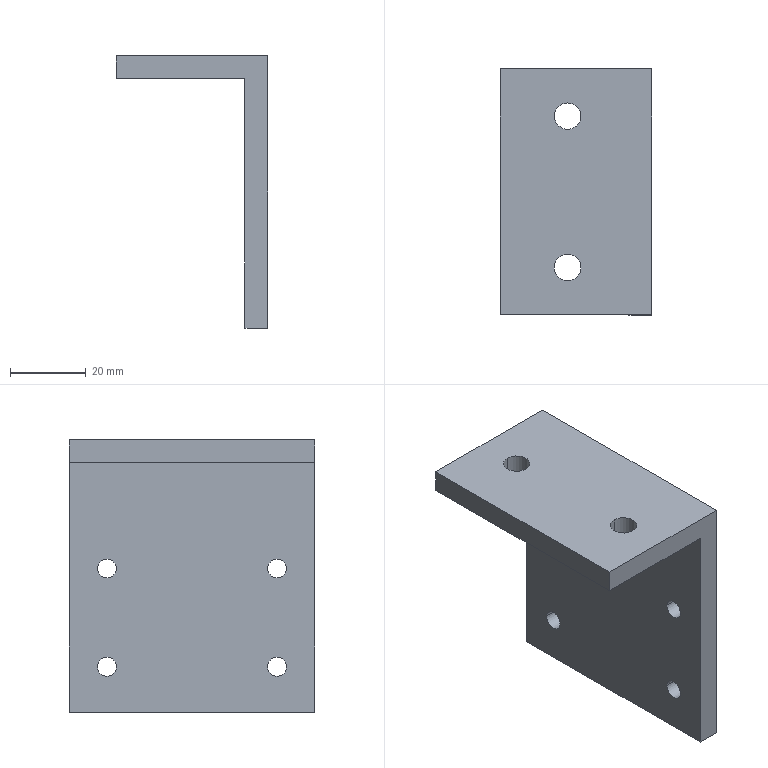Component | SolidWorks | DC-Motor-116-1 | 1 solid | 20 faces | box 40 x 65 x 72 mm | volume 40407 mm3 | cylinder 12 | plane 8 | commonest cylinder face diameters 5 x8 7 x4
build123d program:
from build123d import *

# Parameters (mm, degrees)
BOSS_EXTRUDE1_DEPTH      = 32.5
F_7_0_7_DIAMETER_HOLE1_D = 7
M6_TAPPED_HOLE1_D        = 5


with BuildPart() as part:
    # Sketch1 → Boss-Extrude1 (new, symmetric)
    with BuildSketch(Plane.XY):
        Polygon((-40, 0), (0, 0), (0, 72), (-6, 72), (-6, 6), (-40, 6), align=None)
    extrude(amount=BOSS_EXTRUDE1_DEPTH, both=True)

    # 7.0 _7_ Diameter Hole1 (through all)
    with Locations(Plane(origin=(0, 6, 0), x_dir=(1, 0, 0), z_dir=(0, 1, 0))):
        with Locations((-22.215, 20), (-22.215, -20)):
            Hole(F_7_0_7_DIAMETER_HOLE1_D / 2)

    # M6 Tapped Hole1 (through all)
    with Locations(Plane.ZY.offset(6)):
        with Locations((-22.5, 60), (22.5, 60), (22.5, 34), (-22.5, 34)):
            Hole(M6_TAPPED_HOLE1_D / 2)


solid = part.part

# Placed as in the assembly
solid = solid.moved(Location((-357.792, -173.199, -416), (-90, 0, 0)))
STEP:
#1=COLOUR_RGB('',0.7922,0.8196,0.9333);
#2=FILL_AREA_STYLE_COLOUR('',#1);
#3=FILL_AREA_STYLE('',(#2));
#4=SURFACE_STYLE_FILL_AREA(#3);
#5=SURFACE_SIDE_STYLE('',(#4));
#6=SURFACE_STYLE_USAGE(.BOTH.,#5);
#7=PRESENTATION_STYLE_ASSIGNMENT((#6));
#8=CARTESIAN_POINT('',(-14.086,-7.803,-18.74));
#9=VERTEX_POINT('',#8);
#10=CARTESIAN_POINT('',(-14.086,-7.606,-18.74));
#11=VERTEX_POINT('',#10);
#12=CARTESIAN_POINT('',(-14.086,-7.705,-18.74));
#13=DIRECTION('',(-1.,0.,-0.));
#14=DIRECTION('',(0.,1.,0.));
#15=AXIS2_PLACEMENT_3D('',#12,#13,#14);
#16=CIRCLE('',#15,0.09843);
#17=EDGE_CURVE('',#9,#11,#16,.T.);
#18=ORIENTED_EDGE('',*,*,#17,.F.);
#19=CARTESIAN_POINT('',(-14.323,-7.803,-18.74));
#20=VERTEX_POINT('',#19);
#21=CARTESIAN_POINT('',(-14.323,-7.803,-18.74));
#22=DIRECTION('',(-1.,0.,-0.));
#23=VECTOR('',#22,39.37);
#24=LINE('',#21,#23);
#25=EDGE_CURVE('',#9,#20,#24,.T.);
#26=ORIENTED_EDGE('',*,*,#25,.T.);
#27=CARTESIAN_POINT('',(-14.323,-7.606,-18.74));
#28=VERTEX_POINT('',#27);
#29=CARTESIAN_POINT('',(-14.323,-7.705,-18.74));
#30=DIRECTION('',(-1.,0.,-0.));
#31=DIRECTION('',(0.,1.,0.));
#32=AXIS2_PLACEMENT_3D('',#29,#30,#31);
#33=CIRCLE('',#32,0.09843);
#34=EDGE_CURVE('',#20,#28,#33,.T.);
#35=ORIENTED_EDGE('',*,*,#34,.T.);
#36=CARTESIAN_POINT('',(-14.323,-7.606,-18.74));
#37=DIRECTION('',(-1.,0.,-0.));
#38=VECTOR('',#37,39.37);
#39=LINE('',#36,#38);
#40=EDGE_CURVE('',#11,#28,#39,.T.);
#41=ORIENTED_EDGE('',*,*,#40,.F.);
#42=EDGE_LOOP('',(#18,#26,#35,#41));
#43=FACE_OUTER_BOUND('',#42,.T.);
#44=CARTESIAN_POINT('',(-14.323,-7.705,-18.74));
#45=DIRECTION('',(-1.,0.,-0.));
#46=DIRECTION('',(0.,1.,0.));
#47=AXIS2_PLACEMENT_3D('',#44,#45,#46);
#48=CYLINDRICAL_SURFACE('',#47,0.09843);
#49=ADVANCED_FACE('',(#43),#48,.F.);
#50=CARTESIAN_POINT('',(-14.086,-6.031,-18.74));
#51=VERTEX_POINT('',#50);
#52=CARTESIAN_POINT('',(-14.086,-5.835,-18.74));
#53=VERTEX_POINT('',#52);
#54=CARTESIAN_POINT('',(-14.086,-5.933,-18.74));
#55=DIRECTION('',(-1.,0.,-0.));
#56=DIRECTION('',(0.,1.,0.));
#57=AXIS2_PLACEMENT_3D('',#54,#55,#56);
#58=CIRCLE('',#57,0.09843);
#59=EDGE_CURVE('',#51,#53,#58,.T.);
#60=ORIENTED_EDGE('',*,*,#59,.F.);
#61=CARTESIAN_POINT('',(-14.323,-6.031,-18.74));
#62=VERTEX_POINT('',#61);
#63=CARTESIAN_POINT('',(-14.323,-6.031,-18.74));
#64=DIRECTION('',(-1.,0.,-0.));
#65=VECTOR('',#64,39.37);
#66=LINE('',#63,#65);
#67=EDGE_CURVE('',#51,#62,#66,.T.);
#68=ORIENTED_EDGE('',*,*,#67,.T.);
#69=CARTESIAN_POINT('',(-14.323,-5.835,-18.74));
#70=VERTEX_POINT('',#69);
#71=CARTESIAN_POINT('',(-14.323,-5.933,-18.74));
#72=DIRECTION('',(-1.,0.,-0.));
#73=DIRECTION('',(0.,1.,0.));
#74=AXIS2_PLACEMENT_3D('',#71,#72,#73);
#75=CIRCLE('',#74,0.09843);
#76=EDGE_CURVE('',#62,#70,#75,.T.);
#77=ORIENTED_EDGE('',*,*,#76,.T.);
#78=CARTESIAN_POINT('',(-14.323,-5.835,-18.74));
#79=DIRECTION('',(-1.,0.,-0.));
#80=VECTOR('',#79,39.37);
#81=LINE('',#78,#80);
#82=EDGE_CURVE('',#53,#70,#81,.T.);
#83=ORIENTED_EDGE('',*,*,#82,.F.);
#84=EDGE_LOOP('',(#60,#68,#77,#83));
#85=FACE_OUTER_BOUND('',#84,.T.);
#86=CARTESIAN_POINT('',(-14.323,-5.933,-18.74));
#87=DIRECTION('',(-1.,0.,-0.));
#88=DIRECTION('',(0.,1.,0.));
#89=AXIS2_PLACEMENT_3D('',#86,#87,#88);
#90=CYLINDRICAL_SURFACE('',#89,0.09843);
#91=ADVANCED_FACE('',(#85),#90,.F.);
#92=CARTESIAN_POINT('',(-14.086,-6.031,-17.717));
#93=VERTEX_POINT('',#92);
#94=CARTESIAN_POINT('',(-14.086,-5.835,-17.717));
#95=VERTEX_POINT('',#94);
#96=CARTESIAN_POINT('',(-14.086,-5.933,-17.717));
#97=DIRECTION('',(-1.,0.,-0.));
#98=DIRECTION('',(0.,1.,0.));
#99=AXIS2_PLACEMENT_3D('',#96,#97,#98);
#100=CIRCLE('',#99,0.09843);
#101=EDGE_CURVE('',#93,#95,#100,.T.);
#102=ORIENTED_EDGE('',*,*,#101,.F.);
#103=CARTESIAN_POINT('',(-14.323,-6.031,-17.717));
#104=VERTEX_POINT('',#103);
#105=CARTESIAN_POINT('',(-14.323,-6.031,-17.717));
#106=DIRECTION('',(-1.,0.,-0.));
#107=VECTOR('',#106,39.37);
#108=LINE('',#105,#107);
#109=EDGE_CURVE('',#93,#104,#108,.T.);
#110=ORIENTED_EDGE('',*,*,#109,.T.);
#111=CARTESIAN_POINT('',(-14.323,-5.835,-17.717));
#112=VERTEX_POINT('',#111);
#113=CARTESIAN_POINT('',(-14.323,-5.933,-17.717));
#114=DIRECTION('',(-1.,0.,-0.));
#115=DIRECTION('',(0.,1.,0.));
#116=AXIS2_PLACEMENT_3D('',#113,#114,#115);
#117=CIRCLE('',#116,0.09843);
#118=EDGE_CURVE('',#104,#112,#117,.T.);
#119=ORIENTED_EDGE('',*,*,#118,.T.);
#120=CARTESIAN_POINT('',(-14.323,-5.835,-17.717));
#121=DIRECTION('',(-1.,0.,-0.));
#122=VECTOR('',#121,39.37);
#123=LINE('',#120,#122);
#124=EDGE_CURVE('',#95,#112,#123,.T.);
#125=ORIENTED_EDGE('',*,*,#124,.F.);
#126=EDGE_LOOP('',(#102,#110,#119,#125));
#127=FACE_OUTER_BOUND('',#126,.T.);
#128=CARTESIAN_POINT('',(-14.323,-5.933,-17.717));
#129=DIRECTION('',(-1.,0.,-0.));
#130=DIRECTION('',(0.,1.,0.));
#131=AXIS2_PLACEMENT_3D('',#128,#129,#130);
#132=CYLINDRICAL_SURFACE('',#131,0.09843);
#133=ADVANCED_FACE('',(#127),#132,.F.);
#134=CARTESIAN_POINT('',(-14.086,-7.803,-17.717));
#135=VERTEX_POINT('',#134);
#136=CARTESIAN_POINT('',(-14.086,-7.606,-17.717));
#137=VERTEX_POINT('',#136);
#138=CARTESIAN_POINT('',(-14.086,-7.705,-17.717));
#139=DIRECTION('',(-1.,0.,-0.));
#140=DIRECTION('',(0.,1.,0.));
#141=AXIS2_PLACEMENT_3D('',#138,#139,#140);
#142=CIRCLE('',#141,0.09843);
#143=EDGE_CURVE('',#135,#137,#142,.T.);
#144=ORIENTED_EDGE('',*,*,#143,.F.);
#145=CARTESIAN_POINT('',(-14.323,-7.803,-17.717));
#146=VERTEX_POINT('',#145);
#147=CARTESIAN_POINT('',(-14.323,-7.803,-17.717));
#148=DIRECTION('',(-1.,0.,-0.));
#149=VECTOR('',#148,39.37);
#150=LINE('',#147,#149);
#151=EDGE_CURVE('',#135,#146,#150,.T.);
#152=ORIENTED_EDGE('',*,*,#151,.T.);
#153=CARTESIAN_POINT('',(-14.323,-7.606,-17.717));
#154=VERTEX_POINT('',#153);
#155=CARTESIAN_POINT('',(-14.323,-7.705,-17.717));
#156=DIRECTION('',(-1.,0.,-0.));
#157=DIRECTION('',(0.,1.,0.));
#158=AXIS2_PLACEMENT_3D('',#155,#156,#157);
#159=CIRCLE('',#158,0.09843);
#160=EDGE_CURVE('',#146,#154,#159,.T.);
#161=ORIENTED_EDGE('',*,*,#160,.T.);
#162=CARTESIAN_POINT('',(-14.323,-7.606,-17.717));
#163=DIRECTION('',(-1.,0.,-0.));
#164=VECTOR('',#163,39.37);
#165=LINE('',#162,#164);
#166=EDGE_CURVE('',#137,#154,#165,.T.);
#167=ORIENTED_EDGE('',*,*,#166,.F.);
#168=EDGE_LOOP('',(#144,#152,#161,#167));
#169=FACE_OUTER_BOUND('',#168,.T.);
#170=CARTESIAN_POINT('',(-14.323,-7.705,-17.717));
#171=DIRECTION('',(-1.,0.,-0.));
#172=DIRECTION('',(0.,1.,0.));
#173=AXIS2_PLACEMENT_3D('',#170,#171,#172);
#174=CYLINDRICAL_SURFACE('',#173,0.09843);
#175=ADVANCED_FACE('',(#169),#174,.F.);
#176=CARTESIAN_POINT('',(-14.961,-7.744,-16.378));
#177=VERTEX_POINT('',#176);
#178=CARTESIAN_POINT('',(-14.961,-7.468,-16.378));
#179=VERTEX_POINT('',#178);
#180=CARTESIAN_POINT('',(-14.961,-7.606,-16.378));
#181=DIRECTION('',(0.,0.,-1.));
#182=DIRECTION('',(0.,1.,0.));
#183=AXIS2_PLACEMENT_3D('',#180,#181,#182);
#184=CIRCLE('',#183,0.1378);
#185=EDGE_CURVE('',#177,#179,#184,.T.);
#186=ORIENTED_EDGE('',*,*,#185,.F.);
#187=CARTESIAN_POINT('',(-14.961,-7.744,-16.614));
#188=VERTEX_POINT('',#187);
#189=CARTESIAN_POINT('',(-14.961,-7.744,-16.614));
#190=DIRECTION('',(0.,0.,-1.));
#191=VECTOR('',#190,39.37);
#192=LINE('',#189,#191);
#193=EDGE_CURVE('',#177,#188,#192,.T.);
#194=ORIENTED_EDGE('',*,*,#193,.T.);
#195=CARTESIAN_POINT('',(-14.961,-7.468,-16.614));
#196=VERTEX_POINT('',#195);
#197=CARTESIAN_POINT('',(-14.961,-7.606,-16.614));
#198=DIRECTION('',(0.,0.,-1.));
#199=DIRECTION('',(0.,1.,0.));
#200=AXIS2_PLACEMENT_3D('',#197,#198,#199);
#201=CIRCLE('',#200,0.1378);
#202=EDGE_CURVE('',#188,#196,#201,.T.);
#203=ORIENTED_EDGE('',*,*,#202,.T.);
#204=CARTESIAN_POINT('',(-14.961,-7.468,-16.614));
#205=DIRECTION('',(0.,0.,-1.));
#206=VECTOR('',#205,39.37);
#207=LINE('',#204,#206);
#208=EDGE_CURVE('',#179,#196,#207,.T.);
#209=ORIENTED_EDGE('',*,*,#208,.F.);
#210=EDGE_LOOP('',(#186,#194,#203,#209));
#211=FACE_OUTER_BOUND('',#210,.T.);
#212=CARTESIAN_POINT('',(-14.961,-7.606,-16.614));
#213=DIRECTION('',(0.,0.,-1.));
#214=DIRECTION('',(0.,1.,0.));
#215=AXIS2_PLACEMENT_3D('',#212,#213,#214);
#216=CYLINDRICAL_SURFACE('',#215,0.1378);
#217=ADVANCED_FACE('',(#211),#216,.F.);
#218=CARTESIAN_POINT('',(-14.961,-6.169,-16.378));
#219=VERTEX_POINT('',#218);
#220=CARTESIAN_POINT('',(-14.961,-5.894,-16.378));
#221=VERTEX_POINT('',#220);
#222=CARTESIAN_POINT('',(-14.961,-6.031,-16.378));
#223=DIRECTION('',(0.,0.,-1.));
#224=DIRECTION('',(0.,1.,0.));
#225=AXIS2_PLACEMENT_3D('',#222,#223,#224);
#226=CIRCLE('',#225,0.1378);
#227=EDGE_CURVE('',#219,#221,#226,.T.);
#228=ORIENTED_EDGE('',*,*,#227,.F.);
#229=CARTESIAN_POINT('',(-14.961,-6.169,-16.614));
#230=VERTEX_POINT('',#229);
#231=CARTESIAN_POINT('',(-14.961,-6.169,-16.614));
#232=DIRECTION('',(0.,0.,-1.));
#233=VECTOR('',#232,39.37);
#234=LINE('',#231,#233);
#235=EDGE_CURVE('',#219,#230,#234,.T.);
#236=ORIENTED_EDGE('',*,*,#235,.T.);
#237=CARTESIAN_POINT('',(-14.961,-5.894,-16.614));
#238=VERTEX_POINT('',#237);
#239=CARTESIAN_POINT('',(-14.961,-6.031,-16.614));
#240=DIRECTION('',(0.,0.,-1.));
#241=DIRECTION('',(0.,1.,0.));
#242=AXIS2_PLACEMENT_3D('',#239,#240,#241);
#243=CIRCLE('',#242,0.1378);
#244=EDGE_CURVE('',#230,#238,#243,.T.);
#245=ORIENTED_EDGE('',*,*,#244,.T.);
#246=CARTESIAN_POINT('',(-14.961,-5.894,-16.614));
#247=DIRECTION('',(0.,0.,-1.));
#248=VECTOR('',#247,39.37);
#249=LINE('',#246,#248);
#250=EDGE_CURVE('',#221,#238,#249,.T.);
#251=ORIENTED_EDGE('',*,*,#250,.F.);
#252=EDGE_LOOP('',(#228,#236,#245,#251));
#253=FACE_OUTER_BOUND('',#252,.T.);
#254=CARTESIAN_POINT('',(-14.961,-6.031,-16.614));
#255=DIRECTION('',(0.,0.,-1.));
#256=DIRECTION('',(0.,1.,0.));
#257=AXIS2_PLACEMENT_3D('',#254,#255,#256);
#258=CYLINDRICAL_SURFACE('',#257,0.1378);
#259=ADVANCED_FACE('',(#253),#258,.F.);
#260=CARTESIAN_POINT('',(-15.661,-8.098,-16.614));
#261=VERTEX_POINT('',#260);
#262=CARTESIAN_POINT('',(-15.661,-8.098,-16.378));
#263=VERTEX_POINT('',#262);
#264=CARTESIAN_POINT('',(-15.661,-8.098,-16.614));
#265=DIRECTION('',(-0.,-0.,1.));
#266=VECTOR('',#265,39.37);
#267=LINE('',#264,#266);
#268=EDGE_CURVE('',#261,#263,#267,.T.);
#269=ORIENTED_EDGE('',*,*,#268,.T.);
#270=CARTESIAN_POINT('',(-15.661,-5.539,-16.378));
#271=VERTEX_POINT('',#270);
#272=CARTESIAN_POINT('',(-15.661,-5.539,-16.378));
#273=DIRECTION('',(-0.,-1.,-0.));
#274=VECTOR('',#273,39.37);
#275=LINE('',#272,#274);
#276=EDGE_CURVE('',#271,#263,#275,.T.);
#277=ORIENTED_EDGE('',*,*,#276,.F.);
#278=CARTESIAN_POINT('',(-15.661,-5.539,-16.614));
#279=VERTEX_POINT('',#278);
#280=CARTESIAN_POINT('',(-15.661,-5.539,-16.614));
#281=DIRECTION('',(-0.,-0.,1.));
#282=VECTOR('',#281,39.37);
#283=LINE('',#280,#282);
#284=EDGE_CURVE('',#279,#271,#283,.T.);
#285=ORIENTED_EDGE('',*,*,#284,.F.);
#286=CARTESIAN_POINT('',(-15.661,-5.539,-16.614));
#287=DIRECTION('',(-0.,-1.,-0.));
#288=VECTOR('',#287,39.37);
#289=LINE('',#286,#288);
#290=EDGE_CURVE('',#279,#261,#289,.T.);
#291=ORIENTED_EDGE('',*,*,#290,.T.);
#292=EDGE_LOOP('',(#269,#277,#285,#291));
#293=FACE_OUTER_BOUND('',#292,.T.);
#294=CARTESIAN_POINT('',(-15.661,-5.539,-16.614));
#295=DIRECTION('',(1.,-0.,0.));
#296=DIRECTION('',(-0.,-1.,-0.));
#297=AXIS2_PLACEMENT_3D('',#294,#295,#296);
#298=PLANE('',#297);
#299=ADVANCED_FACE('',(#293),#298,.F.);
#300=CARTESIAN_POINT('',(-14.961,-7.606,-16.378));
#301=DIRECTION('',(0.,0.,-1.));
#302=DIRECTION('',(0.,1.,0.));
#303=AXIS2_PLACEMENT_3D('',#300,#301,#302);
#304=CIRCLE('',#303,0.1378);
#305=EDGE_CURVE('',#179,#177,#304,.T.);
#306=ORIENTED_EDGE('',*,*,#305,.T.);
#307=ORIENTED_EDGE('',*,*,#185,.T.);
#308=EDGE_LOOP('',(#306,#307));
#309=FACE_BOUND('',#308,.T.);
#310=CARTESIAN_POINT('',(-14.961,-6.031,-16.378));
#311=DIRECTION('',(0.,0.,-1.));
#312=DIRECTION('',(0.,1.,0.));
#313=AXIS2_PLACEMENT_3D('',#310,#311,#312);
#314=CIRCLE('',#313,0.1378);
#315=EDGE_CURVE('',#221,#219,#314,.T.);
#316=ORIENTED_EDGE('',*,*,#315,.T.);
#317=ORIENTED_EDGE('',*,*,#227,.T.);
#318=EDGE_LOOP('',(#316,#317));
#319=FACE_BOUND('',#318,.T.);
#320=CARTESIAN_POINT('',(-14.086,-8.098,-16.378));
#321=VERTEX_POINT('',#320);
#322=CARTESIAN_POINT('',(-15.661,-8.098,-16.378));
#323=DIRECTION('',(1.,-0.,0.));
#324=VECTOR('',#323,39.37);
#325=LINE('',#322,#324);
#326=EDGE_CURVE('',#263,#321,#325,.T.);
#327=ORIENTED_EDGE('',*,*,#326,.T.);
#328=CARTESIAN_POINT('',(-14.086,-5.539,-16.378));
#329=VERTEX_POINT('',#328);
#330=CARTESIAN_POINT('',(-14.086,-5.539,-16.378));
#331=DIRECTION('',(-0.,-1.,-0.));
#332=VECTOR('',#331,39.37);
#333=LINE('',#330,#332);
#334=EDGE_CURVE('',#329,#321,#333,.T.);
#335=ORIENTED_EDGE('',*,*,#334,.F.);
#336=CARTESIAN_POINT('',(-15.661,-5.539,-16.378));
#337=DIRECTION('',(1.,-0.,0.));
#338=VECTOR('',#337,39.37);
#339=LINE('',#336,#338);
#340=EDGE_CURVE('',#271,#329,#339,.T.);
#341=ORIENTED_EDGE('',*,*,#340,.F.);
#342=ORIENTED_EDGE('',*,*,#276,.T.);
#343=EDGE_LOOP('',(#327,#335,#341,#342));
#344=FACE_OUTER_BOUND('',#343,.T.);
#345=CARTESIAN_POINT('',(-15.661,-5.539,-16.378));
#346=DIRECTION('',(0.,0.,-1.));
#347=DIRECTION('',(0.,1.,0.));
#348=AXIS2_PLACEMENT_3D('',#345,#346,#347);
#349=PLANE('',#348);
#350=ADVANCED_FACE('',(#309,#319,#344),#349,.F.);
#351=CARTESIAN_POINT('',(-14.086,-7.705,-18.74));
#352=DIRECTION('',(-1.,0.,-0.));
#353=DIRECTION('',(0.,1.,0.));
#354=AXIS2_PLACEMENT_3D('',#351,#352,#353);
#355=CIRCLE('',#354,0.09843);
#356=EDGE_CURVE('',#11,#9,#355,.T.);
#357=ORIENTED_EDGE('',*,*,#356,.T.);
#358=ORIENTED_EDGE('',*,*,#17,.T.);
#359=EDGE_LOOP('',(#357,#358));
#360=FACE_BOUND('',#359,.T.);
#361=CARTESIAN_POINT('',(-14.086,-5.933,-18.74));
#362=DIRECTION('',(-1.,0.,-0.));
#363=DIRECTION('',(0.,1.,0.));
#364=AXIS2_PLACEMENT_3D('',#361,#362,#363);
#365=CIRCLE('',#364,0.09843);
#366=EDGE_CURVE('',#53,#51,#365,.T.);
#367=ORIENTED_EDGE('',*,*,#366,.T.);
#368=ORIENTED_EDGE('',*,*,#59,.T.);
#369=EDGE_LOOP('',(#367,#368));
#370=FACE_BOUND('',#369,.T.);
#371=CARTESIAN_POINT('',(-14.086,-5.933,-17.717));
#372=DIRECTION('',(-1.,0.,-0.));
#373=DIRECTION('',(0.,1.,0.));
#374=AXIS2_PLACEMENT_3D('',#371,#372,#373);
#375=CIRCLE('',#374,0.09843);
#376=EDGE_CURVE('',#95,#93,#375,.T.);
#377=ORIENTED_EDGE('',*,*,#376,.T.);
#378=ORIENTED_EDGE('',*,*,#101,.T.);
#379=EDGE_LOOP('',(#377,#378));
#380=FACE_BOUND('',#379,.T.);
#381=CARTESIAN_POINT('',(-14.086,-7.705,-17.717));
#382=DIRECTION('',(-1.,0.,-0.));
#383=DIRECTION('',(0.,1.,0.));
#384=AXIS2_PLACEMENT_3D('',#381,#382,#383);
#385=CIRCLE('',#384,0.09843);
#386=EDGE_CURVE('',#137,#135,#385,.T.);
#387=ORIENTED_EDGE('',*,*,#386,.T.);
#388=ORIENTED_EDGE('',*,*,#143,.T.);
#389=EDGE_LOOP('',(#387,#388));
#390=FACE_BOUND('',#389,.T.);
#391=CARTESIAN_POINT('',(-14.086,-8.098,-19.213));
#392=VERTEX_POINT('',#391);
#393=CARTESIAN_POINT('',(-14.086,-8.098,-16.378));
#394=DIRECTION('',(0.,0.,-1.));
#395=VECTOR('',#394,39.37);
#396=LINE('',#393,#395);
#397=EDGE_CURVE('',#321,#392,#396,.T.);
#398=ORIENTED_EDGE('',*,*,#397,.T.);
#399=CARTESIAN_POINT('',(-14.086,-5.539,-19.213));
#400=VERTEX_POINT('',#399);
#401=CARTESIAN_POINT('',(-14.086,-5.539,-19.213));
#402=DIRECTION('',(-0.,-1.,-0.));
#403=VECTOR('',#402,39.37);
#404=LINE('',#401,#403);
#405=EDGE_CURVE('',#400,#392,#404,.T.);
#406=ORIENTED_EDGE('',*,*,#405,.F.);
#407=CARTESIAN_POINT('',(-14.086,-5.539,-16.378));
#408=DIRECTION('',(0.,0.,-1.));
#409=VECTOR('',#408,39.37);
#410=LINE('',#407,#409);
#411=EDGE_CURVE('',#329,#400,#410,.T.);
#412=ORIENTED_EDGE('',*,*,#411,.F.);
#413=ORIENTED_EDGE('',*,*,#334,.T.);
#414=EDGE_LOOP('',(#398,#406,#412,#413));
#415=FACE_OUTER_BOUND('',#414,.T.);
#416=CARTESIAN_POINT('',(-14.086,-5.539,-16.378));
#417=DIRECTION('',(-1.,0.,-0.));
#418=DIRECTION('',(0.,1.,0.));
#419=AXIS2_PLACEMENT_3D('',#416,#417,#418);
#420=PLANE('',#419);
#421=ADVANCED_FACE('',(#360,#370,#380,#390,#415),#420,.F.);
#422=CARTESIAN_POINT('',(-14.323,-8.098,-19.213));
#423=VERTEX_POINT('',#422);
#424=CARTESIAN_POINT('',(-14.323,-8.098,-19.213));
#425=DIRECTION('',(-1.,0.,-0.));
#426=VECTOR('',#425,39.37);
#427=LINE('',#424,#426);
#428=EDGE_CURVE('',#392,#423,#427,.T.);
#429=ORIENTED_EDGE('',*,*,#428,.T.);
#430=CARTESIAN_POINT('',(-14.323,-5.539,-19.213));
#431=VERTEX_POINT('',#430);
#432=CARTESIAN_POINT('',(-14.323,-5.539,-19.213));
#433=DIRECTION('',(-0.,-1.,-0.));
#434=VECTOR('',#433,39.37);
#435=LINE('',#432,#434);
#436=EDGE_CURVE('',#431,#423,#435,.T.);
#437=ORIENTED_EDGE('',*,*,#436,.F.);
#438=CARTESIAN_POINT('',(-14.323,-5.539,-19.213));
#439=DIRECTION('',(-1.,0.,-0.));
#440=VECTOR('',#439,39.37);
#441=LINE('',#438,#440);
#442=EDGE_CURVE('',#400,#431,#441,.T.);
#443=ORIENTED_EDGE('',*,*,#442,.F.);
#444=ORIENTED_EDGE('',*,*,#405,.T.);
#445=EDGE_LOOP('',(#429,#437,#443,#444));
#446=FACE_OUTER_BOUND('',#445,.T.);
#447=CARTESIAN_POINT('',(-14.323,-5.539,-19.213));
#448=DIRECTION('',(-0.,-0.,1.));
#449=DIRECTION('',(-0.,-1.,-0.));
#450=AXIS2_PLACEMENT_3D('',#447,#448,#449);
#451=PLANE('',#450);
#452=ADVANCED_FACE('',(#446),#451,.F.);
#453=CARTESIAN_POINT('',(-14.323,-7.705,-18.74));
#454=DIRECTION('',(-1.,0.,-0.));
#455=DIRECTION('',(0.,1.,0.));
#456=AXIS2_PLACEMENT_3D('',#453,#454,#455);
#457=CIRCLE('',#456,0.09843);
#458=EDGE_CURVE('',#28,#20,#457,.T.);
#459=ORIENTED_EDGE('',*,*,#458,.F.);
#460=ORIENTED_EDGE('',*,*,#34,.F.);
#461=EDGE_LOOP('',(#459,#460));
#462=FACE_BOUND('',#461,.T.);
#463=CARTESIAN_POINT('',(-14.323,-5.933,-18.74));
#464=DIRECTION('',(-1.,0.,-0.));
#465=DIRECTION('',(0.,1.,0.));
#466=AXIS2_PLACEMENT_3D('',#463,#464,#465);
#467=CIRCLE('',#466,0.09843);
#468=EDGE_CURVE('',#70,#62,#467,.T.);
#469=ORIENTED_EDGE('',*,*,#468,.F.);
#470=ORIENTED_EDGE('',*,*,#76,.F.);
#471=EDGE_LOOP('',(#469,#470));
#472=FACE_BOUND('',#471,.T.);
#473=CARTESIAN_POINT('',(-14.323,-5.933,-17.717));
#474=DIRECTION('',(-1.,0.,-0.));
#475=DIRECTION('',(0.,1.,0.));
#476=AXIS2_PLACEMENT_3D('',#473,#474,#475);
#477=CIRCLE('',#476,0.09843);
#478=EDGE_CURVE('',#112,#104,#477,.T.);
#479=ORIENTED_EDGE('',*,*,#478,.F.);
#480=ORIENTED_EDGE('',*,*,#118,.F.);
#481=EDGE_LOOP('',(#479,#480));
#482=FACE_BOUND('',#481,.T.);
#483=CARTESIAN_POINT('',(-14.323,-7.705,-17.717));
#484=DIRECTION('',(-1.,0.,-0.));
#485=DIRECTION('',(0.,1.,0.));
#486=AXIS2_PLACEMENT_3D('',#483,#484,#485);
#487=CIRCLE('',#486,0.09843);
#488=EDGE_CURVE('',#154,#146,#487,.T.);
#489=ORIENTED_EDGE('',*,*,#488,.F.);
#490=ORIENTED_EDGE('',*,*,#160,.F.);
#491=EDGE_LOOP('',(#489,#490));
#492=FACE_BOUND('',#491,.T.);
#493=CARTESIAN_POINT('',(-14.323,-8.098,-16.614));
#494=VERTEX_POINT('',#493);
#495=CARTESIAN_POINT('',(-14.323,-8.098,-16.614));
#496=DIRECTION('',(-0.,-0.,1.));
#497=VECTOR('',#496,39.37);
#498=LINE('',#495,#497);
#499=EDGE_CURVE('',#423,#494,#498,.T.);
#500=ORIENTED_EDGE('',*,*,#499,.T.);
#501=CARTESIAN_POINT('',(-14.323,-5.539,-16.614));
#502=VERTEX_POINT('',#501);
#503=CARTESIAN_POINT('',(-14.323,-5.539,-16.614));
#504=DIRECTION('',(-0.,-1.,-0.));
#505=VECTOR('',#504,39.37);
#506=LINE('',#503,#505);
#507=EDGE_CURVE('',#502,#494,#506,.T.);
#508=ORIENTED_EDGE('',*,*,#507,.F.);
#509=CARTESIAN_POINT('',(-14.323,-5.539,-16.614));
#510=DIRECTION('',(-0.,-0.,1.));
#511=VECTOR('',#510,39.37);
#512=LINE('',#509,#511);
#513=EDGE_CURVE('',#431,#502,#512,.T.);
#514=ORIENTED_EDGE('',*,*,#513,.F.);
#515=ORIENTED_EDGE('',*,*,#436,.T.);
#516=EDGE_LOOP('',(#500,#508,#514,#515));
#517=FACE_OUTER_BOUND('',#516,.T.);
#518=CARTESIAN_POINT('',(-14.323,-5.539,-16.614));
#519=DIRECTION('',(1.,-0.,0.));
#520=DIRECTION('',(-0.,-1.,-0.));
#521=AXIS2_PLACEMENT_3D('',#518,#519,#520);
#522=PLANE('',#521);
#523=ADVANCED_FACE('',(#462,#472,#482,#492,#517),#522,.F.);
#524=CARTESIAN_POINT('',(-14.961,-7.606,-16.614));
#525=DIRECTION('',(0.,0.,-1.));
#526=DIRECTION('',(0.,1.,0.));
#527=AXIS2_PLACEMENT_3D('',#524,#525,#526);
#528=CIRCLE('',#527,0.1378);
#529=EDGE_CURVE('',#196,#188,#528,.T.);
#530=ORIENTED_EDGE('',*,*,#529,.F.);
#531=ORIENTED_EDGE('',*,*,#202,.F.);
#532=EDGE_LOOP('',(#530,#531));
#533=FACE_BOUND('',#532,.T.);
#534=CARTESIAN_POINT('',(-14.961,-6.031,-16.614));
#535=DIRECTION('',(0.,0.,-1.));
#536=DIRECTION('',(0.,1.,0.));
#537=AXIS2_PLACEMENT_3D('',#534,#535,#536);
#538=CIRCLE('',#537,0.1378);
#539=EDGE_CURVE('',#238,#230,#538,.T.);
#540=ORIENTED_EDGE('',*,*,#539,.F.);
#541=ORIENTED_EDGE('',*,*,#244,.F.);
#542=EDGE_LOOP('',(#540,#541));
#543=FACE_BOUND('',#542,.T.);
#544=CARTESIAN_POINT('',(-15.661,-8.098,-16.614));
#545=DIRECTION('',(-1.,0.,-0.));
#546=VECTOR('',#545,39.37);
#547=LINE('',#544,#546);
#548=EDGE_CURVE('',#494,#261,#547,.T.);
#549=ORIENTED_EDGE('',*,*,#548,.T.);
#550=ORIENTED_EDGE('',*,*,#290,.F.);
#551=CARTESIAN_POINT('',(-15.661,-5.539,-16.614));
#552=DIRECTION('',(-1.,0.,-0.));
#553=VECTOR('',#552,39.37);
#554=LINE('',#551,#553);
#555=EDGE_CURVE('',#502,#279,#554,.T.);
#556=ORIENTED_EDGE('',*,*,#555,.F.);
#557=ORIENTED_EDGE('',*,*,#507,.T.);
#558=EDGE_LOOP('',(#549,#550,#556,#557));
#559=FACE_OUTER_BOUND('',#558,.T.);
#560=CARTESIAN_POINT('',(-15.661,-5.539,-16.614));
#561=DIRECTION('',(-0.,-0.,1.));
#562=DIRECTION('',(-0.,-1.,-0.));
#563=AXIS2_PLACEMENT_3D('',#560,#561,#562);
#564=PLANE('',#563);
#565=ADVANCED_FACE('',(#533,#543,#559),#564,.F.);
#566=ORIENTED_EDGE('',*,*,#284,.T.);
#567=ORIENTED_EDGE('',*,*,#340,.T.);
#568=ORIENTED_EDGE('',*,*,#411,.T.);
#569=ORIENTED_EDGE('',*,*,#442,.T.);
#570=ORIENTED_EDGE('',*,*,#513,.T.);
#571=ORIENTED_EDGE('',*,*,#555,.T.);
#572=EDGE_LOOP('',(#566,#567,#568,#569,#570,#571));
#573=FACE_OUTER_BOUND('',#572,.T.);
#574=CARTESIAN_POINT('',(-14.086,-5.539,-16.378));
#575=DIRECTION('',(0.,1.,0.));
#576=DIRECTION('',(1.,-0.,0.));
#577=AXIS2_PLACEMENT_3D('',#574,#575,#576);
#578=PLANE('',#577);
#579=ADVANCED_FACE('',(#573),#578,.T.);
#580=ORIENTED_EDGE('',*,*,#268,.F.);
#581=ORIENTED_EDGE('',*,*,#548,.F.);
#582=ORIENTED_EDGE('',*,*,#499,.F.);
#583=ORIENTED_EDGE('',*,*,#428,.F.);
#584=ORIENTED_EDGE('',*,*,#397,.F.);
#585=ORIENTED_EDGE('',*,*,#326,.F.);
#586=EDGE_LOOP('',(#580,#581,#582,#583,#584,#585));
#587=FACE_OUTER_BOUND('',#586,.T.);
#588=CARTESIAN_POINT('',(-14.086,-8.098,-16.378));
#589=DIRECTION('',(0.,1.,0.));
#590=DIRECTION('',(1.,-0.,0.));
#591=AXIS2_PLACEMENT_3D('',#588,#589,#590);
#592=PLANE('',#591);
#593=ADVANCED_FACE('',(#587),#592,.F.);
#594=ORIENTED_EDGE('',*,*,#235,.F.);
#595=ORIENTED_EDGE('',*,*,#315,.F.);
#596=ORIENTED_EDGE('',*,*,#250,.T.);
#597=ORIENTED_EDGE('',*,*,#539,.T.);
#598=EDGE_LOOP('',(#594,#595,#596,#597));
#599=FACE_OUTER_BOUND('',#598,.T.);
#600=CARTESIAN_POINT('',(-14.961,-6.031,-16.614));
#601=DIRECTION('',(0.,0.,-1.));
#602=DIRECTION('',(0.,1.,0.));
#603=AXIS2_PLACEMENT_3D('',#600,#601,#602);
#604=CYLINDRICAL_SURFACE('',#603,0.1378);
#605=ADVANCED_FACE('',(#599),#604,.F.);
#606=ORIENTED_EDGE('',*,*,#193,.F.);
#607=ORIENTED_EDGE('',*,*,#305,.F.);
#608=ORIENTED_EDGE('',*,*,#208,.T.);
#609=ORIENTED_EDGE('',*,*,#529,.T.);
#610=EDGE_LOOP('',(#606,#607,#608,#609));
#611=FACE_OUTER_BOUND('',#610,.T.);
#612=CARTESIAN_POINT('',(-14.961,-7.606,-16.614));
#613=DIRECTION('',(0.,0.,-1.));
#614=DIRECTION('',(0.,1.,0.));
#615=AXIS2_PLACEMENT_3D('',#612,#613,#614);
#616=CYLINDRICAL_SURFACE('',#615,0.1378);
#617=ADVANCED_FACE('',(#611),#616,.F.);
#618=ORIENTED_EDGE('',*,*,#151,.F.);
#619=ORIENTED_EDGE('',*,*,#386,.F.);
#620=ORIENTED_EDGE('',*,*,#166,.T.);
#621=ORIENTED_EDGE('',*,*,#488,.T.);
#622=EDGE_LOOP('',(#618,#619,#620,#621));
#623=FACE_OUTER_BOUND('',#622,.T.);
#624=CARTESIAN_POINT('',(-14.323,-7.705,-17.717));
#625=DIRECTION('',(-1.,0.,-0.));
#626=DIRECTION('',(0.,1.,0.));
#627=AXIS2_PLACEMENT_3D('',#624,#625,#626);
#628=CYLINDRICAL_SURFACE('',#627,0.09843);
#629=ADVANCED_FACE('',(#623),#628,.F.);
#630=ORIENTED_EDGE('',*,*,#109,.F.);
#631=ORIENTED_EDGE('',*,*,#376,.F.);
#632=ORIENTED_EDGE('',*,*,#124,.T.);
#633=ORIENTED_EDGE('',*,*,#478,.T.);
#634=EDGE_LOOP('',(#630,#631,#632,#633));
#635=FACE_OUTER_BOUND('',#634,.T.);
#636=CARTESIAN_POINT('',(-14.323,-5.933,-17.717));
#637=DIRECTION('',(-1.,0.,-0.));
#638=DIRECTION('',(0.,1.,0.));
#639=AXIS2_PLACEMENT_3D('',#636,#637,#638);
#640=CYLINDRICAL_SURFACE('',#639,0.09843);
#641=ADVANCED_FACE('',(#635),#640,.F.);
#642=ORIENTED_EDGE('',*,*,#67,.F.);
#643=ORIENTED_EDGE('',*,*,#366,.F.);
#644=ORIENTED_EDGE('',*,*,#82,.T.);
#645=ORIENTED_EDGE('',*,*,#468,.T.);
#646=EDGE_LOOP('',(#642,#643,#644,#645));
#647=FACE_OUTER_BOUND('',#646,.T.);
#648=CARTESIAN_POINT('',(-14.323,-5.933,-18.74));
#649=DIRECTION('',(-1.,0.,-0.));
#650=DIRECTION('',(0.,1.,0.));
#651=AXIS2_PLACEMENT_3D('',#648,#649,#650);
#652=CYLINDRICAL_SURFACE('',#651,0.09843);
#653=ADVANCED_FACE('',(#647),#652,.F.);
#654=ORIENTED_EDGE('',*,*,#25,.F.);
#655=ORIENTED_EDGE('',*,*,#356,.F.);
#656=ORIENTED_EDGE('',*,*,#40,.T.);
#657=ORIENTED_EDGE('',*,*,#458,.T.);
#658=EDGE_LOOP('',(#654,#655,#656,#657));
#659=FACE_OUTER_BOUND('',#658,.T.);
#660=CARTESIAN_POINT('',(-14.323,-7.705,-18.74));
#661=DIRECTION('',(-1.,0.,-0.));
#662=DIRECTION('',(0.,1.,0.));
#663=AXIS2_PLACEMENT_3D('',#660,#661,#662);
#664=CYLINDRICAL_SURFACE('',#663,0.09843);
#665=ADVANCED_FACE('',(#659),#664,.F.);
#666=CLOSED_SHELL('',(#49,#91,#133,#175,#217,#259,#299,#350,#421,#452,#523,#565,#579,#593,#605,#617,#629,#641,#653,#665));
#667=MANIFOLD_SOLID_BREP('',#666);
#668=STYLED_ITEM('',(#7),#667);
#669=(LENGTH_UNIT()NAMED_UNIT(*)SI_UNIT($,.METRE.));
#670=LENGTH_MEASURE_WITH_UNIT(LENGTH_MEASURE(0.0254),#669);
#671=DIMENSIONAL_EXPONENTS(1.,0.,0.,0.,0.,0.,0.);
#672=(CONVERSION_BASED_UNIT('',#670)LENGTH_UNIT()NAMED_UNIT(#671));
#673=UNCERTAINTY_MEASURE_WITH_UNIT(LENGTH_MEASURE(0.00001),#672,'','');
#674=(NAMED_UNIT(*)PLANE_ANGLE_UNIT()SI_UNIT($,.RADIAN.));
#675=(NAMED_UNIT(*)SI_UNIT($,.STERADIAN.)SOLID_ANGLE_UNIT());
#676=(GEOMETRIC_REPRESENTATION_CONTEXT(3)GLOBAL_UNCERTAINTY_ASSIGNED_CONTEXT((#673))GLOBAL_UNIT_ASSIGNED_CONTEXT((#672,#674,#675))REPRESENTATION_CONTEXT('',''));
#677=MECHANICAL_DESIGN_GEOMETRIC_PRESENTATION_REPRESENTATION('',(#668),#676);
#678=PRESENTATION_LAYER_ASSIGNMENT('','',(#668));
#679=CARTESIAN_POINT('',(0.,0.,0.));
#680=DIRECTION('',(0.,0.,1.));
#681=DIRECTION('',(1.,0.,0.));
#682=AXIS2_PLACEMENT_3D('',#679,#680,#681);
#683=(LENGTH_UNIT()NAMED_UNIT(*)SI_UNIT($,.METRE.));
#684=LENGTH_MEASURE_WITH_UNIT(LENGTH_MEASURE(0.0254),#683);
#685=DIMENSIONAL_EXPONENTS(1.,0.,0.,0.,0.,0.,0.);
#686=(CONVERSION_BASED_UNIT('',#684)LENGTH_UNIT()NAMED_UNIT(#685));
#687=UNCERTAINTY_MEASURE_WITH_UNIT(LENGTH_MEASURE(0.00001),#686,'','');
#688=(NAMED_UNIT(*)PLANE_ANGLE_UNIT()SI_UNIT($,.RADIAN.));
#689=(NAMED_UNIT(*)SI_UNIT($,.STERADIAN.)SOLID_ANGLE_UNIT());
#690=(GEOMETRIC_REPRESENTATION_CONTEXT(3)GLOBAL_UNCERTAINTY_ASSIGNED_CONTEXT((#687))GLOBAL_UNIT_ASSIGNED_CONTEXT((#686,#688,#689))REPRESENTATION_CONTEXT('',''));
#691=ADVANCED_BREP_SHAPE_REPRESENTATION('',(#667,#682),#690);